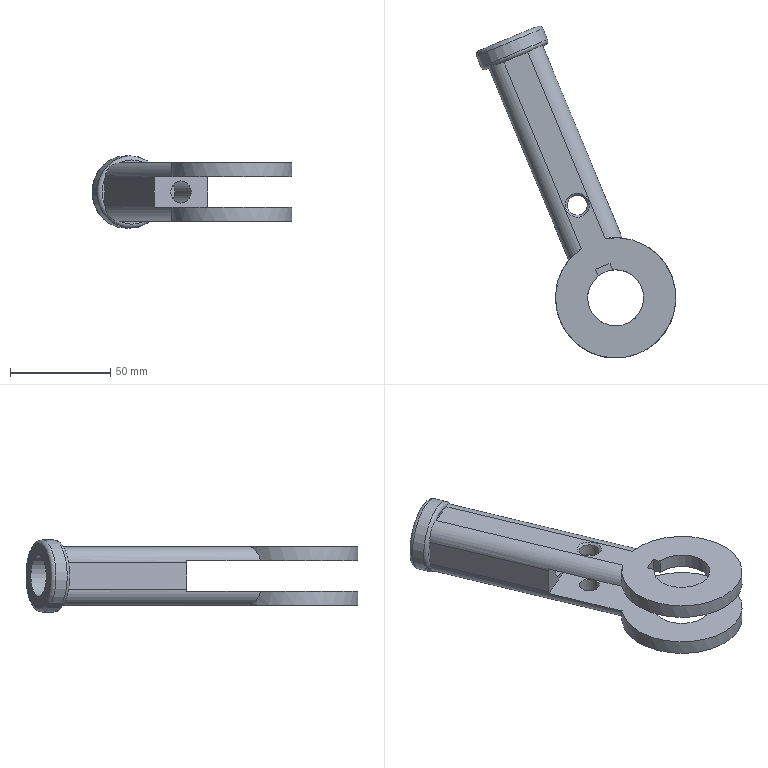Component | NX | HANDLESLEEVE | 1 solid | 34 faces | volume 90036 mm3 | plane 16 | cylinder 14 | torus 2 | cone 2 | commonest cylinder face diameters 16 x4 28 x2 60 x2 10 x2 36 x1 20 x1 5 x1 11 x1